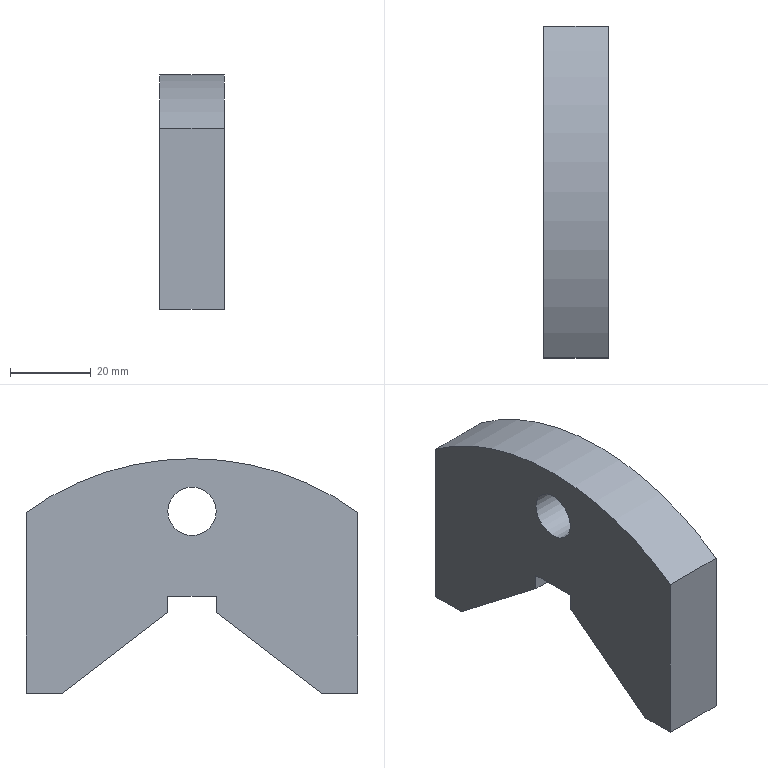Component | NX | V_BLOCK | 1 solid | 13 faces | box 16 x 82 x 58 mm | volume 55776 mm3 | plane 11 | cylinder 2 | commonest cylinder face diameters 140 x1 12 x1
STEP:
#1=CARTESIAN_POINT('',(0.,0.,0.));
#2=DIRECTION('',(0.,0.,1.));
#3=DIRECTION('',(1.,0.,0.));
#4=AXIS2_PLACEMENT_3D('',#1,#2,#3);
#5=CARTESIAN_POINT('',(47.,-41.,189.249));
#6=VERTEX_POINT('',#5);
#7=CARTESIAN_POINT('',(47.,-41.,144.513));
#8=VERTEX_POINT('',#7);
#9=CARTESIAN_POINT('',(47.,-41.,189.249));
#10=DIRECTION('',(0.,-0.,-1.));
#11=VECTOR('',#10,1.);
#12=LINE('',#9,#11);
#13=CARTESIAN_POINT('',(63.,-41.,189.249));
#14=DIRECTION('',(0.,1.,-0.));
#15=DIRECTION('',(0.,0.,1.));
#16=AXIS2_PLACEMENT_3D('',#13,#14,#15);
#17=PLANE('',#16);
#18=CARTESIAN_POINT('',(0.,-16.));
#19=DIRECTION('',(-1.,0.));
#20=VECTOR('',#19,1.);
#21=LINE('',#18,#20);
#22=(GEOMETRIC_REPRESENTATION_CONTEXT(2)PARAMETRIC_REPRESENTATION_CONTEXT()REPRESENTATION_CONTEXT('',''));
#23=DEFINITIONAL_REPRESENTATION('',(#21),#22);
#24=PCURVE('',#17,#23);
#25=CARTESIAN_POINT('',(47.,0.,132.513));
#26=DIRECTION('',(1.,0.,0.));
#27=DIRECTION('',(0.,0.,-1.));
#28=AXIS2_PLACEMENT_3D('',#25,#26,#27);
#29=PLANE('',#28);
#30=CARTESIAN_POINT('',(-56.736,-41.));
#31=DIRECTION('',(1.,-0.));
#32=VECTOR('',#31,1.);
#33=LINE('',#30,#32);
#34=(GEOMETRIC_REPRESENTATION_CONTEXT(2)PARAMETRIC_REPRESENTATION_CONTEXT()REPRESENTATION_CONTEXT('',''));
#35=DEFINITIONAL_REPRESENTATION('',(#33),#34);
#36=PCURVE('',#29,#35);
#37=SURFACE_CURVE('',#12,(#24,#36),.PCURVE_S1.);
#38=EDGE_CURVE('',#6,#8,#37,.T.);
#39=ORIENTED_EDGE('',*,*,#38,.T.);
#40=CARTESIAN_POINT('',(63.,-41.,144.513));
#41=VERTEX_POINT('',#40);
#42=CARTESIAN_POINT('',(63.,-41.,144.513));
#43=DIRECTION('',(-1.,0.,0.));
#44=VECTOR('',#43,1.);
#45=LINE('',#42,#44);
#46=CARTESIAN_POINT('',(-44.736,0.));
#47=DIRECTION('',(0.,-1.));
#48=VECTOR('',#47,1.);
#49=LINE('',#46,#48);
#50=(GEOMETRIC_REPRESENTATION_CONTEXT(2)PARAMETRIC_REPRESENTATION_CONTEXT()REPRESENTATION_CONTEXT('',''));
#51=DEFINITIONAL_REPRESENTATION('',(#49),#50);
#52=PCURVE('',#17,#51);
#53=CARTESIAN_POINT('',(63.,-41.,144.513));
#54=DIRECTION('',(0.,0.,1.));
#55=DIRECTION('',(0.,-1.,0.));
#56=AXIS2_PLACEMENT_3D('',#53,#54,#55);
#57=PLANE('',#56);
#58=CARTESIAN_POINT('',(0.,0.));
#59=DIRECTION('',(0.,-1.));
#60=VECTOR('',#59,1.);
#61=LINE('',#58,#60);
#62=(GEOMETRIC_REPRESENTATION_CONTEXT(2)PARAMETRIC_REPRESENTATION_CONTEXT()REPRESENTATION_CONTEXT('',''));
#63=DEFINITIONAL_REPRESENTATION('',(#61),#62);
#64=PCURVE('',#57,#63);
#65=SURFACE_CURVE('',#45,(#52,#64),.PCURVE_S1.);
#66=EDGE_CURVE('',#41,#8,#65,.T.);
#67=ORIENTED_EDGE('',*,*,#66,.F.);
#68=CARTESIAN_POINT('',(63.,-41.,189.249));
#69=VERTEX_POINT('',#68);
#70=CARTESIAN_POINT('',(63.,-41.,189.249));
#71=DIRECTION('',(0.,-0.,-1.));
#72=VECTOR('',#71,1.);
#73=LINE('',#70,#72);
#74=CARTESIAN_POINT('',(0.,0.));
#75=DIRECTION('',(-1.,0.));
#76=VECTOR('',#75,1.);
#77=LINE('',#74,#76);
#78=(GEOMETRIC_REPRESENTATION_CONTEXT(2)PARAMETRIC_REPRESENTATION_CONTEXT()REPRESENTATION_CONTEXT('',''));
#79=DEFINITIONAL_REPRESENTATION('',(#77),#78);
#80=PCURVE('',#17,#79);
#81=CARTESIAN_POINT('',(63.,0.,132.513));
#82=DIRECTION('',(1.,0.,0.));
#83=DIRECTION('',(0.,0.,-1.));
#84=AXIS2_PLACEMENT_3D('',#81,#82,#83);
#85=PLANE('',#84);
#86=CARTESIAN_POINT('',(-56.736,-41.));
#87=DIRECTION('',(1.,-0.));
#88=VECTOR('',#87,1.);
#89=LINE('',#86,#88);
#90=(GEOMETRIC_REPRESENTATION_CONTEXT(2)PARAMETRIC_REPRESENTATION_CONTEXT()REPRESENTATION_CONTEXT('',''));
#91=DEFINITIONAL_REPRESENTATION('',(#89),#90);
#92=PCURVE('',#85,#91);
#93=SURFACE_CURVE('',#73,(#80,#92),.PCURVE_S1.);
#94=EDGE_CURVE('',#69,#41,#93,.T.);
#95=ORIENTED_EDGE('',*,*,#94,.F.);
#96=CARTESIAN_POINT('',(63.,-41.,189.249));
#97=DIRECTION('',(-1.,0.,0.));
#98=VECTOR('',#97,1.);
#99=LINE('',#96,#98);
#100=CARTESIAN_POINT('',(0.,0.));
#101=DIRECTION('',(0.,-1.));
#102=VECTOR('',#101,1.);
#103=LINE('',#100,#102);
#104=(GEOMETRIC_REPRESENTATION_CONTEXT(2)PARAMETRIC_REPRESENTATION_CONTEXT()REPRESENTATION_CONTEXT('',''));
#105=DEFINITIONAL_REPRESENTATION('',(#103),#104);
#106=PCURVE('',#17,#105);
#107=CARTESIAN_POINT('',(63.,0.,132.513));
#108=DIRECTION('',(-1.,0.,0.));
#109=DIRECTION('',(0.,0.,1.));
#110=AXIS2_PLACEMENT_3D('',#107,#108,#109);
#111=CYLINDRICAL_SURFACE('',#110,70.);
#112=CARTESIAN_POINT('',(-0.6258,0.));
#113=DIRECTION('',(0.,1.));
#114=VECTOR('',#113,1.);
#115=LINE('',#112,#114);
#116=(GEOMETRIC_REPRESENTATION_CONTEXT(2)PARAMETRIC_REPRESENTATION_CONTEXT()REPRESENTATION_CONTEXT('',''));
#117=DEFINITIONAL_REPRESENTATION('',(#115),#116);
#118=PCURVE('',#111,#117);
#119=SURFACE_CURVE('',#99,(#106,#118),.PCURVE_S1.);
#120=EDGE_CURVE('',#69,#6,#119,.T.);
#121=ORIENTED_EDGE('',*,*,#120,.T.);
#122=EDGE_LOOP('',(#39,#67,#95,#121));
#123=FACE_BOUND('',#122,.T.);
#124=ADVANCED_FACE('',(#123),#17,.F.);
#125=CARTESIAN_POINT('',(47.,-32.065,144.513));
#126=VERTEX_POINT('',#125);
#127=CARTESIAN_POINT('',(47.,-41.,144.513));
#128=DIRECTION('',(0.,1.,-0.));
#129=VECTOR('',#128,1.);
#130=LINE('',#127,#129);
#131=CARTESIAN_POINT('',(0.,-16.));
#132=DIRECTION('',(-1.,0.));
#133=VECTOR('',#132,1.);
#134=LINE('',#131,#133);
#135=(GEOMETRIC_REPRESENTATION_CONTEXT(2)PARAMETRIC_REPRESENTATION_CONTEXT()REPRESENTATION_CONTEXT('',''));
#136=DEFINITIONAL_REPRESENTATION('',(#134),#135);
#137=PCURVE('',#57,#136);
#138=CARTESIAN_POINT('',(-12.,-41.));
#139=DIRECTION('',(0.,1.));
#140=VECTOR('',#139,1.);
#141=LINE('',#138,#140);
#142=(GEOMETRIC_REPRESENTATION_CONTEXT(2)PARAMETRIC_REPRESENTATION_CONTEXT()REPRESENTATION_CONTEXT('',''));
#143=DEFINITIONAL_REPRESENTATION('',(#141),#142);
#144=PCURVE('',#29,#143);
#145=SURFACE_CURVE('',#130,(#137,#144),.PCURVE_S1.);
#146=EDGE_CURVE('',#8,#126,#145,.T.);
#147=ORIENTED_EDGE('',*,*,#146,.T.);
#148=CARTESIAN_POINT('',(63.,-32.065,144.513));
#149=VERTEX_POINT('',#148);
#150=CARTESIAN_POINT('',(63.,-32.065,144.513));
#151=DIRECTION('',(-1.,0.,0.));
#152=VECTOR('',#151,1.);
#153=LINE('',#150,#152);
#154=CARTESIAN_POINT('',(-8.935,0.));
#155=DIRECTION('',(0.,-1.));
#156=VECTOR('',#155,1.);
#157=LINE('',#154,#156);
#158=(GEOMETRIC_REPRESENTATION_CONTEXT(2)PARAMETRIC_REPRESENTATION_CONTEXT()REPRESENTATION_CONTEXT('',''));
#159=DEFINITIONAL_REPRESENTATION('',(#157),#158);
#160=PCURVE('',#57,#159);
#161=CARTESIAN_POINT('',(63.,-32.065,144.513));
#162=DIRECTION('',(0.,-0.6088,0.7934));
#163=DIRECTION('',(0.,-0.7934,-0.6088));
#164=AXIS2_PLACEMENT_3D('',#161,#162,#163);
#165=PLANE('',#164);
#166=CARTESIAN_POINT('',(0.,0.));
#167=DIRECTION('',(0.,-1.));
#168=VECTOR('',#167,1.);
#169=LINE('',#166,#168);
#170=(GEOMETRIC_REPRESENTATION_CONTEXT(2)PARAMETRIC_REPRESENTATION_CONTEXT()REPRESENTATION_CONTEXT('',''));
#171=DEFINITIONAL_REPRESENTATION('',(#169),#170);
#172=PCURVE('',#165,#171);
#173=SURFACE_CURVE('',#153,(#160,#172),.PCURVE_S1.);
#174=EDGE_CURVE('',#149,#126,#173,.T.);
#175=ORIENTED_EDGE('',*,*,#174,.F.);
#176=CARTESIAN_POINT('',(63.,-41.,144.513));
#177=DIRECTION('',(0.,1.,-0.));
#178=VECTOR('',#177,1.);
#179=LINE('',#176,#178);
#180=CARTESIAN_POINT('',(0.,0.));
#181=DIRECTION('',(-1.,0.));
#182=VECTOR('',#181,1.);
#183=LINE('',#180,#182);
#184=(GEOMETRIC_REPRESENTATION_CONTEXT(2)PARAMETRIC_REPRESENTATION_CONTEXT()REPRESENTATION_CONTEXT('',''));
#185=DEFINITIONAL_REPRESENTATION('',(#183),#184);
#186=PCURVE('',#57,#185);
#187=CARTESIAN_POINT('',(-12.,-41.));
#188=DIRECTION('',(0.,1.));
#189=VECTOR('',#188,1.);
#190=LINE('',#187,#189);
#191=(GEOMETRIC_REPRESENTATION_CONTEXT(2)PARAMETRIC_REPRESENTATION_CONTEXT()REPRESENTATION_CONTEXT('',''));
#192=DEFINITIONAL_REPRESENTATION('',(#190),#191);
#193=PCURVE('',#85,#192);
#194=SURFACE_CURVE('',#179,(#186,#193),.PCURVE_S1.);
#195=EDGE_CURVE('',#41,#149,#194,.T.);
#196=ORIENTED_EDGE('',*,*,#195,.F.);
#197=ORIENTED_EDGE('',*,*,#66,.T.);
#198=EDGE_LOOP('',(#147,#175,#196,#197));
#199=FACE_BOUND('',#198,.T.);
#200=ADVANCED_FACE('',(#199),#57,.F.);
#201=CARTESIAN_POINT('',(47.,-6.,164.513));
#202=VERTEX_POINT('',#201);
#203=CARTESIAN_POINT('',(47.,-32.065,144.513));
#204=DIRECTION('',(0.,0.7934,0.6088));
#205=VECTOR('',#204,1.);
#206=LINE('',#203,#205);
#207=CARTESIAN_POINT('',(0.,-16.));
#208=DIRECTION('',(-1.,0.));
#209=VECTOR('',#208,1.);
#210=LINE('',#207,#209);
#211=(GEOMETRIC_REPRESENTATION_CONTEXT(2)PARAMETRIC_REPRESENTATION_CONTEXT()REPRESENTATION_CONTEXT('',''));
#212=DEFINITIONAL_REPRESENTATION('',(#210),#211);
#213=PCURVE('',#165,#212);
#214=CARTESIAN_POINT('',(-12.,-32.065));
#215=DIRECTION('',(-0.6088,0.7934));
#216=VECTOR('',#215,1.);
#217=LINE('',#214,#216);
#218=(GEOMETRIC_REPRESENTATION_CONTEXT(2)PARAMETRIC_REPRESENTATION_CONTEXT()REPRESENTATION_CONTEXT('',''));
#219=DEFINITIONAL_REPRESENTATION('',(#217),#218);
#220=PCURVE('',#29,#219);
#221=SURFACE_CURVE('',#206,(#213,#220),.PCURVE_S1.);
#222=EDGE_CURVE('',#126,#202,#221,.T.);
#223=ORIENTED_EDGE('',*,*,#222,.T.);
#224=CARTESIAN_POINT('',(63.,-6.,164.513));
#225=VERTEX_POINT('',#224);
#226=CARTESIAN_POINT('',(63.,-6.,164.513));
#227=DIRECTION('',(-1.,0.,0.));
#228=VECTOR('',#227,1.);
#229=LINE('',#226,#228);
#230=CARTESIAN_POINT('',(-32.854,0.));
#231=DIRECTION('',(0.,-1.));
#232=VECTOR('',#231,1.);
#233=LINE('',#230,#232);
#234=(GEOMETRIC_REPRESENTATION_CONTEXT(2)PARAMETRIC_REPRESENTATION_CONTEXT()REPRESENTATION_CONTEXT('',''));
#235=DEFINITIONAL_REPRESENTATION('',(#233),#234);
#236=PCURVE('',#165,#235);
#237=CARTESIAN_POINT('',(63.,-6.,164.513));
#238=DIRECTION('',(0.,-1.,0.));
#239=DIRECTION('',(0.,0.,-1.));
#240=AXIS2_PLACEMENT_3D('',#237,#238,#239);
#241=PLANE('',#240);
#242=CARTESIAN_POINT('',(0.,0.));
#243=DIRECTION('',(0.,-1.));
#244=VECTOR('',#243,1.);
#245=LINE('',#242,#244);
#246=(GEOMETRIC_REPRESENTATION_CONTEXT(2)PARAMETRIC_REPRESENTATION_CONTEXT()REPRESENTATION_CONTEXT('',''));
#247=DEFINITIONAL_REPRESENTATION('',(#245),#246);
#248=PCURVE('',#241,#247);
#249=SURFACE_CURVE('',#229,(#236,#248),.PCURVE_S1.);
#250=EDGE_CURVE('',#225,#202,#249,.T.);
#251=ORIENTED_EDGE('',*,*,#250,.F.);
#252=CARTESIAN_POINT('',(63.,-32.065,144.513));
#253=DIRECTION('',(0.,0.7934,0.6088));
#254=VECTOR('',#253,1.);
#255=LINE('',#252,#254);
#256=CARTESIAN_POINT('',(0.,0.));
#257=DIRECTION('',(-1.,0.));
#258=VECTOR('',#257,1.);
#259=LINE('',#256,#258);
#260=(GEOMETRIC_REPRESENTATION_CONTEXT(2)PARAMETRIC_REPRESENTATION_CONTEXT()REPRESENTATION_CONTEXT('',''));
#261=DEFINITIONAL_REPRESENTATION('',(#259),#260);
#262=PCURVE('',#165,#261);
#263=CARTESIAN_POINT('',(-12.,-32.065));
#264=DIRECTION('',(-0.6088,0.7934));
#265=VECTOR('',#264,1.);
#266=LINE('',#263,#265);
#267=(GEOMETRIC_REPRESENTATION_CONTEXT(2)PARAMETRIC_REPRESENTATION_CONTEXT()REPRESENTATION_CONTEXT('',''));
#268=DEFINITIONAL_REPRESENTATION('',(#266),#267);
#269=PCURVE('',#85,#268);
#270=SURFACE_CURVE('',#255,(#262,#269),.PCURVE_S1.);
#271=EDGE_CURVE('',#149,#225,#270,.T.);
#272=ORIENTED_EDGE('',*,*,#271,.F.);
#273=ORIENTED_EDGE('',*,*,#174,.T.);
#274=EDGE_LOOP('',(#223,#251,#272,#273));
#275=FACE_BOUND('',#274,.T.);
#276=ADVANCED_FACE('',(#275),#165,.F.);
#277=CARTESIAN_POINT('',(47.,-6.,168.513));
#278=VERTEX_POINT('',#277);
#279=CARTESIAN_POINT('',(47.,-6.,164.513));
#280=DIRECTION('',(0.,0.,1.));
#281=VECTOR('',#280,1.);
#282=LINE('',#279,#281);
#283=CARTESIAN_POINT('',(0.,-16.));
#284=DIRECTION('',(-1.,0.));
#285=VECTOR('',#284,1.);
#286=LINE('',#283,#285);
#287=(GEOMETRIC_REPRESENTATION_CONTEXT(2)PARAMETRIC_REPRESENTATION_CONTEXT()REPRESENTATION_CONTEXT('',''));
#288=DEFINITIONAL_REPRESENTATION('',(#286),#287);
#289=PCURVE('',#241,#288);
#290=CARTESIAN_POINT('',(-32.,-6.));
#291=DIRECTION('',(-1.,0.));
#292=VECTOR('',#291,1.);
#293=LINE('',#290,#292);
#294=(GEOMETRIC_REPRESENTATION_CONTEXT(2)PARAMETRIC_REPRESENTATION_CONTEXT()REPRESENTATION_CONTEXT('',''));
#295=DEFINITIONAL_REPRESENTATION('',(#293),#294);
#296=PCURVE('',#29,#295);
#297=SURFACE_CURVE('',#282,(#289,#296),.PCURVE_S1.);
#298=EDGE_CURVE('',#202,#278,#297,.T.);
#299=ORIENTED_EDGE('',*,*,#298,.T.);
#300=CARTESIAN_POINT('',(63.,-6.,168.513));
#301=VERTEX_POINT('',#300);
#302=CARTESIAN_POINT('',(63.,-6.,168.513));
#303=DIRECTION('',(-1.,0.,0.));
#304=VECTOR('',#303,1.);
#305=LINE('',#302,#304);
#306=CARTESIAN_POINT('',(-4.,0.));
#307=DIRECTION('',(0.,-1.));
#308=VECTOR('',#307,1.);
#309=LINE('',#306,#308);
#310=(GEOMETRIC_REPRESENTATION_CONTEXT(2)PARAMETRIC_REPRESENTATION_CONTEXT()REPRESENTATION_CONTEXT('',''));
#311=DEFINITIONAL_REPRESENTATION('',(#309),#310);
#312=PCURVE('',#241,#311);
#313=CARTESIAN_POINT('',(63.,0.,168.513));
#314=DIRECTION('',(0.,0.,1.));
#315=DIRECTION('',(1.,0.,0.));
#316=AXIS2_PLACEMENT_3D('',#313,#314,#315);
#317=PLANE('',#316);
#318=CARTESIAN_POINT('',(0.,-6.));
#319=DIRECTION('',(-1.,0.));
#320=VECTOR('',#319,1.);
#321=LINE('',#318,#320);
#322=(GEOMETRIC_REPRESENTATION_CONTEXT(2)PARAMETRIC_REPRESENTATION_CONTEXT()REPRESENTATION_CONTEXT('',''));
#323=DEFINITIONAL_REPRESENTATION('',(#321),#322);
#324=PCURVE('',#317,#323);
#325=SURFACE_CURVE('',#305,(#312,#324),.PCURVE_S1.);
#326=EDGE_CURVE('',#301,#278,#325,.T.);
#327=ORIENTED_EDGE('',*,*,#326,.F.);
#328=CARTESIAN_POINT('',(63.,-6.,164.513));
#329=DIRECTION('',(0.,0.,1.));
#330=VECTOR('',#329,1.);
#331=LINE('',#328,#330);
#332=CARTESIAN_POINT('',(0.,0.));
#333=DIRECTION('',(-1.,0.));
#334=VECTOR('',#333,1.);
#335=LINE('',#332,#334);
#336=(GEOMETRIC_REPRESENTATION_CONTEXT(2)PARAMETRIC_REPRESENTATION_CONTEXT()REPRESENTATION_CONTEXT('',''));
#337=DEFINITIONAL_REPRESENTATION('',(#335),#336);
#338=PCURVE('',#241,#337);
#339=CARTESIAN_POINT('',(-32.,-6.));
#340=DIRECTION('',(-1.,0.));
#341=VECTOR('',#340,1.);
#342=LINE('',#339,#341);
#343=(GEOMETRIC_REPRESENTATION_CONTEXT(2)PARAMETRIC_REPRESENTATION_CONTEXT()REPRESENTATION_CONTEXT('',''));
#344=DEFINITIONAL_REPRESENTATION('',(#342),#343);
#345=PCURVE('',#85,#344);
#346=SURFACE_CURVE('',#331,(#338,#345),.PCURVE_S1.);
#347=EDGE_CURVE('',#225,#301,#346,.T.);
#348=ORIENTED_EDGE('',*,*,#347,.F.);
#349=ORIENTED_EDGE('',*,*,#250,.T.);
#350=EDGE_LOOP('',(#299,#327,#348,#349));
#351=FACE_BOUND('',#350,.T.);
#352=ADVANCED_FACE('',(#351),#241,.F.);
#353=CARTESIAN_POINT('',(47.,6.,168.513));
#354=VERTEX_POINT('',#353);
#355=CARTESIAN_POINT('',(47.,0.,168.513));
#356=DIRECTION('',(0.,1.,0.));
#357=VECTOR('',#356,1.);
#358=LINE('',#355,#357);
#359=CARTESIAN_POINT('',(-16.,0.));
#360=DIRECTION('',(0.,1.));
#361=VECTOR('',#360,1.);
#362=LINE('',#359,#361);
#363=(GEOMETRIC_REPRESENTATION_CONTEXT(2)PARAMETRIC_REPRESENTATION_CONTEXT()REPRESENTATION_CONTEXT('',''));
#364=DEFINITIONAL_REPRESENTATION('',(#362),#363);
#365=PCURVE('',#317,#364);
#366=CARTESIAN_POINT('',(-36.,0.));
#367=DIRECTION('',(0.,1.));
#368=VECTOR('',#367,1.);
#369=LINE('',#366,#368);
#370=(GEOMETRIC_REPRESENTATION_CONTEXT(2)PARAMETRIC_REPRESENTATION_CONTEXT()REPRESENTATION_CONTEXT('',''));
#371=DEFINITIONAL_REPRESENTATION('',(#369),#370);
#372=PCURVE('',#29,#371);
#373=SURFACE_CURVE('',#358,(#365,#372),.PCURVE_S1.);
#374=EDGE_CURVE('',#278,#354,#373,.T.);
#375=ORIENTED_EDGE('',*,*,#374,.T.);
#376=CARTESIAN_POINT('',(63.,6.,168.513));
#377=VERTEX_POINT('',#376);
#378=CARTESIAN_POINT('',(63.,6.,168.513));
#379=DIRECTION('',(-1.,0.,0.));
#380=VECTOR('',#379,1.);
#381=LINE('',#378,#380);
#382=CARTESIAN_POINT('',(0.,6.));
#383=DIRECTION('',(-1.,0.));
#384=VECTOR('',#383,1.);
#385=LINE('',#382,#384);
#386=(GEOMETRIC_REPRESENTATION_CONTEXT(2)PARAMETRIC_REPRESENTATION_CONTEXT()REPRESENTATION_CONTEXT('',''));
#387=DEFINITIONAL_REPRESENTATION('',(#385),#386);
#388=PCURVE('',#317,#387);
#389=CARTESIAN_POINT('',(63.,6.,168.513));
#390=DIRECTION('',(0.,1.,0.));
#391=DIRECTION('',(0.,0.,1.));
#392=AXIS2_PLACEMENT_3D('',#389,#390,#391);
#393=PLANE('',#392);
#394=CARTESIAN_POINT('',(0.,0.));
#395=DIRECTION('',(0.,-1.));
#396=VECTOR('',#395,1.);
#397=LINE('',#394,#396);
#398=(GEOMETRIC_REPRESENTATION_CONTEXT(2)PARAMETRIC_REPRESENTATION_CONTEXT()REPRESENTATION_CONTEXT('',''));
#399=DEFINITIONAL_REPRESENTATION('',(#397),#398);
#400=PCURVE('',#393,#399);
#401=SURFACE_CURVE('',#381,(#388,#400),.PCURVE_S1.);
#402=EDGE_CURVE('',#377,#354,#401,.T.);
#403=ORIENTED_EDGE('',*,*,#402,.F.);
#404=CARTESIAN_POINT('',(63.,-6.,168.513));
#405=DIRECTION('',(0.,1.,0.));
#406=VECTOR('',#405,1.);
#407=LINE('',#404,#406);
#408=CARTESIAN_POINT('',(0.,-6.));
#409=DIRECTION('',(0.,1.));
#410=VECTOR('',#409,1.);
#411=LINE('',#408,#410);
#412=(GEOMETRIC_REPRESENTATION_CONTEXT(2)PARAMETRIC_REPRESENTATION_CONTEXT()REPRESENTATION_CONTEXT('',''));
#413=DEFINITIONAL_REPRESENTATION('',(#411),#412);
#414=PCURVE('',#317,#413);
#415=CARTESIAN_POINT('',(-36.,-6.));
#416=DIRECTION('',(0.,1.));
#417=VECTOR('',#416,1.);
#418=LINE('',#415,#417);
#419=(GEOMETRIC_REPRESENTATION_CONTEXT(2)PARAMETRIC_REPRESENTATION_CONTEXT()REPRESENTATION_CONTEXT('',''));
#420=DEFINITIONAL_REPRESENTATION('',(#418),#419);
#421=PCURVE('',#85,#420);
#422=SURFACE_CURVE('',#407,(#414,#421),.PCURVE_S1.);
#423=EDGE_CURVE('',#301,#377,#422,.T.);
#424=ORIENTED_EDGE('',*,*,#423,.F.);
#425=ORIENTED_EDGE('',*,*,#326,.T.);
#426=EDGE_LOOP('',(#375,#403,#424,#425));
#427=FACE_BOUND('',#426,.T.);
#428=ADVANCED_FACE('',(#427),#317,.F.);
#429=CARTESIAN_POINT('',(47.,6.,164.513));
#430=VERTEX_POINT('',#429);
#431=CARTESIAN_POINT('',(47.,6.,168.513));
#432=DIRECTION('',(0.,0.,-1.));
#433=VECTOR('',#432,1.);
#434=LINE('',#431,#433);
#435=CARTESIAN_POINT('',(0.,-16.));
#436=DIRECTION('',(-1.,0.));
#437=VECTOR('',#436,1.);
#438=LINE('',#435,#437);
#439=(GEOMETRIC_REPRESENTATION_CONTEXT(2)PARAMETRIC_REPRESENTATION_CONTEXT()REPRESENTATION_CONTEXT('',''));
#440=DEFINITIONAL_REPRESENTATION('',(#438),#439);
#441=PCURVE('',#393,#440);
#442=CARTESIAN_POINT('',(-36.,6.));
#443=DIRECTION('',(1.,0.));
#444=VECTOR('',#443,1.);
#445=LINE('',#442,#444);
#446=(GEOMETRIC_REPRESENTATION_CONTEXT(2)PARAMETRIC_REPRESENTATION_CONTEXT()REPRESENTATION_CONTEXT('',''));
#447=DEFINITIONAL_REPRESENTATION('',(#445),#446);
#448=PCURVE('',#29,#447);
#449=SURFACE_CURVE('',#434,(#441,#448),.PCURVE_S1.);
#450=EDGE_CURVE('',#354,#430,#449,.T.);
#451=ORIENTED_EDGE('',*,*,#450,.T.);
#452=CARTESIAN_POINT('',(63.,6.,164.513));
#453=VERTEX_POINT('',#452);
#454=CARTESIAN_POINT('',(63.,6.,164.513));
#455=DIRECTION('',(-1.,0.,0.));
#456=VECTOR('',#455,1.);
#457=LINE('',#454,#456);
#458=CARTESIAN_POINT('',(-4.,0.));
#459=DIRECTION('',(0.,-1.));
#460=VECTOR('',#459,1.);
#461=LINE('',#458,#460);
#462=(GEOMETRIC_REPRESENTATION_CONTEXT(2)PARAMETRIC_REPRESENTATION_CONTEXT()REPRESENTATION_CONTEXT('',''));
#463=DEFINITIONAL_REPRESENTATION('',(#461),#462);
#464=PCURVE('',#393,#463);
#465=CARTESIAN_POINT('',(63.,6.,164.513));
#466=DIRECTION('',(0.,0.6088,0.7934));
#467=DIRECTION('',(0.,-0.7934,0.6088));
#468=AXIS2_PLACEMENT_3D('',#465,#466,#467);
#469=PLANE('',#468);
#470=CARTESIAN_POINT('',(0.,0.));
#471=DIRECTION('',(0.,-1.));
#472=VECTOR('',#471,1.);
#473=LINE('',#470,#472);
#474=(GEOMETRIC_REPRESENTATION_CONTEXT(2)PARAMETRIC_REPRESENTATION_CONTEXT()REPRESENTATION_CONTEXT('',''));
#475=DEFINITIONAL_REPRESENTATION('',(#473),#474);
#476=PCURVE('',#469,#475);
#477=SURFACE_CURVE('',#457,(#464,#476),.PCURVE_S1.);
#478=EDGE_CURVE('',#453,#430,#477,.T.);
#479=ORIENTED_EDGE('',*,*,#478,.F.);
#480=CARTESIAN_POINT('',(63.,6.,168.513));
#481=DIRECTION('',(0.,0.,-1.));
#482=VECTOR('',#481,1.);
#483=LINE('',#480,#482);
#484=CARTESIAN_POINT('',(0.,0.));
#485=DIRECTION('',(-1.,0.));
#486=VECTOR('',#485,1.);
#487=LINE('',#484,#486);
#488=(GEOMETRIC_REPRESENTATION_CONTEXT(2)PARAMETRIC_REPRESENTATION_CONTEXT()REPRESENTATION_CONTEXT('',''));
#489=DEFINITIONAL_REPRESENTATION('',(#487),#488);
#490=PCURVE('',#393,#489);
#491=CARTESIAN_POINT('',(-36.,6.));
#492=DIRECTION('',(1.,0.));
#493=VECTOR('',#492,1.);
#494=LINE('',#491,#493);
#495=(GEOMETRIC_REPRESENTATION_CONTEXT(2)PARAMETRIC_REPRESENTATION_CONTEXT()REPRESENTATION_CONTEXT('',''));
#496=DEFINITIONAL_REPRESENTATION('',(#494),#495);
#497=PCURVE('',#85,#496);
#498=SURFACE_CURVE('',#483,(#490,#497),.PCURVE_S1.);
#499=EDGE_CURVE('',#377,#453,#498,.T.);
#500=ORIENTED_EDGE('',*,*,#499,.F.);
#501=ORIENTED_EDGE('',*,*,#402,.T.);
#502=EDGE_LOOP('',(#451,#479,#500,#501));
#503=FACE_BOUND('',#502,.T.);
#504=ADVANCED_FACE('',(#503),#393,.F.);
#505=CARTESIAN_POINT('',(47.,32.065,144.513));
#506=VERTEX_POINT('',#505);
#507=CARTESIAN_POINT('',(47.,6.,164.513));
#508=DIRECTION('',(0.,0.7934,-0.6088));
#509=VECTOR('',#508,1.);
#510=LINE('',#507,#509);
#511=CARTESIAN_POINT('',(0.,-16.));
#512=DIRECTION('',(-1.,0.));
#513=VECTOR('',#512,1.);
#514=LINE('',#511,#513);
#515=(GEOMETRIC_REPRESENTATION_CONTEXT(2)PARAMETRIC_REPRESENTATION_CONTEXT()REPRESENTATION_CONTEXT('',''));
#516=DEFINITIONAL_REPRESENTATION('',(#514),#515);
#517=PCURVE('',#469,#516);
#518=CARTESIAN_POINT('',(-32.,6.));
#519=DIRECTION('',(0.6088,0.7934));
#520=VECTOR('',#519,1.);
#521=LINE('',#518,#520);
#522=(GEOMETRIC_REPRESENTATION_CONTEXT(2)PARAMETRIC_REPRESENTATION_CONTEXT()REPRESENTATION_CONTEXT('',''));
#523=DEFINITIONAL_REPRESENTATION('',(#521),#522);
#524=PCURVE('',#29,#523);
#525=SURFACE_CURVE('',#510,(#517,#524),.PCURVE_S1.);
#526=EDGE_CURVE('',#430,#506,#525,.T.);
#527=ORIENTED_EDGE('',*,*,#526,.T.);
#528=CARTESIAN_POINT('',(63.,32.065,144.513));
#529=VERTEX_POINT('',#528);
#530=CARTESIAN_POINT('',(63.,32.065,144.513));
#531=DIRECTION('',(-1.,0.,0.));
#532=VECTOR('',#531,1.);
#533=LINE('',#530,#532);
#534=CARTESIAN_POINT('',(-32.854,0.));
#535=DIRECTION('',(0.,-1.));
#536=VECTOR('',#535,1.);
#537=LINE('',#534,#536);
#538=(GEOMETRIC_REPRESENTATION_CONTEXT(2)PARAMETRIC_REPRESENTATION_CONTEXT()REPRESENTATION_CONTEXT('',''));
#539=DEFINITIONAL_REPRESENTATION('',(#537),#538);
#540=PCURVE('',#469,#539);
#541=CARTESIAN_POINT('',(63.,32.065,144.513));
#542=DIRECTION('',(0.,-0.,1.));
#543=DIRECTION('',(0.,-1.,-0.));
#544=AXIS2_PLACEMENT_3D('',#541,#542,#543);
#545=PLANE('',#544);
#546=CARTESIAN_POINT('',(0.,0.));
#547=DIRECTION('',(0.,-1.));
#548=VECTOR('',#547,1.);
#549=LINE('',#546,#548);
#550=(GEOMETRIC_REPRESENTATION_CONTEXT(2)PARAMETRIC_REPRESENTATION_CONTEXT()REPRESENTATION_CONTEXT('',''));
#551=DEFINITIONAL_REPRESENTATION('',(#549),#550);
#552=PCURVE('',#545,#551);
#553=SURFACE_CURVE('',#533,(#540,#552),.PCURVE_S1.);
#554=EDGE_CURVE('',#529,#506,#553,.T.);
#555=ORIENTED_EDGE('',*,*,#554,.F.);
#556=CARTESIAN_POINT('',(63.,6.,164.513));
#557=DIRECTION('',(0.,0.7934,-0.6088));
#558=VECTOR('',#557,1.);
#559=LINE('',#556,#558);
#560=CARTESIAN_POINT('',(0.,0.));
#561=DIRECTION('',(-1.,0.));
#562=VECTOR('',#561,1.);
#563=LINE('',#560,#562);
#564=(GEOMETRIC_REPRESENTATION_CONTEXT(2)PARAMETRIC_REPRESENTATION_CONTEXT()REPRESENTATION_CONTEXT('',''));
#565=DEFINITIONAL_REPRESENTATION('',(#563),#564);
#566=PCURVE('',#469,#565);
#567=CARTESIAN_POINT('',(-32.,6.));
#568=DIRECTION('',(0.6088,0.7934));
#569=VECTOR('',#568,1.);
#570=LINE('',#567,#569);
#571=(GEOMETRIC_REPRESENTATION_CONTEXT(2)PARAMETRIC_REPRESENTATION_CONTEXT()REPRESENTATION_CONTEXT('',''));
#572=DEFINITIONAL_REPRESENTATION('',(#570),#571);
#573=PCURVE('',#85,#572);
#574=SURFACE_CURVE('',#559,(#566,#573),.PCURVE_S1.);
#575=EDGE_CURVE('',#453,#529,#574,.T.);
#576=ORIENTED_EDGE('',*,*,#575,.F.);
#577=ORIENTED_EDGE('',*,*,#478,.T.);
#578=EDGE_LOOP('',(#527,#555,#576,#577));
#579=FACE_BOUND('',#578,.T.);
#580=ADVANCED_FACE('',(#579),#469,.F.);
#581=CARTESIAN_POINT('',(47.,41.,144.513));
#582=VERTEX_POINT('',#581);
#583=CARTESIAN_POINT('',(47.,32.065,144.513));
#584=DIRECTION('',(0.,1.,0.));
#585=VECTOR('',#584,1.);
#586=LINE('',#583,#585);
#587=CARTESIAN_POINT('',(0.,-16.));
#588=DIRECTION('',(-1.,0.));
#589=VECTOR('',#588,1.);
#590=LINE('',#587,#589);
#591=(GEOMETRIC_REPRESENTATION_CONTEXT(2)PARAMETRIC_REPRESENTATION_CONTEXT()REPRESENTATION_CONTEXT('',''));
#592=DEFINITIONAL_REPRESENTATION('',(#590),#591);
#593=PCURVE('',#545,#592);
#594=CARTESIAN_POINT('',(-12.,32.065));
#595=DIRECTION('',(-0.,1.));
#596=VECTOR('',#595,1.);
#597=LINE('',#594,#596);
#598=(GEOMETRIC_REPRESENTATION_CONTEXT(2)PARAMETRIC_REPRESENTATION_CONTEXT()REPRESENTATION_CONTEXT('',''));
#599=DEFINITIONAL_REPRESENTATION('',(#597),#598);
#600=PCURVE('',#29,#599);
#601=SURFACE_CURVE('',#586,(#593,#600),.PCURVE_S1.);
#602=EDGE_CURVE('',#506,#582,#601,.T.);
#603=ORIENTED_EDGE('',*,*,#602,.T.);
#604=CARTESIAN_POINT('',(63.,41.,144.513));
#605=VERTEX_POINT('',#604);
#606=CARTESIAN_POINT('',(63.,41.,144.513));
#607=DIRECTION('',(-1.,0.,0.));
#608=VECTOR('',#607,1.);
#609=LINE('',#606,#608);
#610=CARTESIAN_POINT('',(-8.935,0.));
#611=DIRECTION('',(0.,-1.));
#612=VECTOR('',#611,1.);
#613=LINE('',#610,#612);
#614=(GEOMETRIC_REPRESENTATION_CONTEXT(2)PARAMETRIC_REPRESENTATION_CONTEXT()REPRESENTATION_CONTEXT('',''));
#615=DEFINITIONAL_REPRESENTATION('',(#613),#614);
#616=PCURVE('',#545,#615);
#617=CARTESIAN_POINT('',(63.,41.,144.513));
#618=DIRECTION('',(0.,-1.,-0.));
#619=DIRECTION('',(0.,0.,-1.));
#620=AXIS2_PLACEMENT_3D('',#617,#618,#619);
#621=PLANE('',#620);
#622=CARTESIAN_POINT('',(0.,0.));
#623=DIRECTION('',(0.,-1.));
#624=VECTOR('',#623,1.);
#625=LINE('',#622,#624);
#626=(GEOMETRIC_REPRESENTATION_CONTEXT(2)PARAMETRIC_REPRESENTATION_CONTEXT()REPRESENTATION_CONTEXT('',''));
#627=DEFINITIONAL_REPRESENTATION('',(#625),#626);
#628=PCURVE('',#621,#627);
#629=SURFACE_CURVE('',#609,(#616,#628),.PCURVE_S1.);
#630=EDGE_CURVE('',#605,#582,#629,.T.);
#631=ORIENTED_EDGE('',*,*,#630,.F.);
#632=CARTESIAN_POINT('',(63.,32.065,144.513));
#633=DIRECTION('',(0.,1.,0.));
#634=VECTOR('',#633,1.);
#635=LINE('',#632,#634);
#636=CARTESIAN_POINT('',(0.,0.));
#637=DIRECTION('',(-1.,0.));
#638=VECTOR('',#637,1.);
#639=LINE('',#636,#638);
#640=(GEOMETRIC_REPRESENTATION_CONTEXT(2)PARAMETRIC_REPRESENTATION_CONTEXT()REPRESENTATION_CONTEXT('',''));
#641=DEFINITIONAL_REPRESENTATION('',(#639),#640);
#642=PCURVE('',#545,#641);
#643=CARTESIAN_POINT('',(-12.,32.065));
#644=DIRECTION('',(-0.,1.));
#645=VECTOR('',#644,1.);
#646=LINE('',#643,#645);
#647=(GEOMETRIC_REPRESENTATION_CONTEXT(2)PARAMETRIC_REPRESENTATION_CONTEXT()REPRESENTATION_CONTEXT('',''));
#648=DEFINITIONAL_REPRESENTATION('',(#646),#647);
#649=PCURVE('',#85,#648);
#650=SURFACE_CURVE('',#635,(#642,#649),.PCURVE_S1.);
#651=EDGE_CURVE('',#529,#605,#650,.T.);
#652=ORIENTED_EDGE('',*,*,#651,.F.);
#653=ORIENTED_EDGE('',*,*,#554,.T.);
#654=EDGE_LOOP('',(#603,#631,#652,#653));
#655=FACE_BOUND('',#654,.T.);
#656=ADVANCED_FACE('',(#655),#545,.F.);
#657=CARTESIAN_POINT('',(47.,41.,189.249));
#658=VERTEX_POINT('',#657);
#659=CARTESIAN_POINT('',(47.,41.,144.513));
#660=DIRECTION('',(0.,-0.,1.));
#661=VECTOR('',#660,1.);
#662=LINE('',#659,#661);
#663=CARTESIAN_POINT('',(0.,-16.));
#664=DIRECTION('',(-1.,0.));
#665=VECTOR('',#664,1.);
#666=LINE('',#663,#665);
#667=(GEOMETRIC_REPRESENTATION_CONTEXT(2)PARAMETRIC_REPRESENTATION_CONTEXT()REPRESENTATION_CONTEXT('',''));
#668=DEFINITIONAL_REPRESENTATION('',(#666),#667);
#669=PCURVE('',#621,#668);
#670=CARTESIAN_POINT('',(-12.,41.));
#671=DIRECTION('',(-1.,-0.));
#672=VECTOR('',#671,1.);
#673=LINE('',#670,#672);
#674=(GEOMETRIC_REPRESENTATION_CONTEXT(2)PARAMETRIC_REPRESENTATION_CONTEXT()REPRESENTATION_CONTEXT('',''));
#675=DEFINITIONAL_REPRESENTATION('',(#673),#674);
#676=PCURVE('',#29,#675);
#677=SURFACE_CURVE('',#662,(#669,#676),.PCURVE_S1.);
#678=EDGE_CURVE('',#582,#658,#677,.T.);
#679=ORIENTED_EDGE('',*,*,#678,.T.);
#680=CARTESIAN_POINT('',(63.,41.,189.249));
#681=VERTEX_POINT('',#680);
#682=CARTESIAN_POINT('',(63.,41.,189.249));
#683=DIRECTION('',(-1.,0.,0.));
#684=VECTOR('',#683,1.);
#685=LINE('',#682,#684);
#686=CARTESIAN_POINT('',(-44.736,0.));
#687=DIRECTION('',(0.,-1.));
#688=VECTOR('',#687,1.);
#689=LINE('',#686,#688);
#690=(GEOMETRIC_REPRESENTATION_CONTEXT(2)PARAMETRIC_REPRESENTATION_CONTEXT()REPRESENTATION_CONTEXT('',''));
#691=DEFINITIONAL_REPRESENTATION('',(#689),#690);
#692=PCURVE('',#621,#691);
#693=CARTESIAN_POINT('',(0.6258,0.));
#694=DIRECTION('',(0.,1.));
#695=VECTOR('',#694,1.);
#696=LINE('',#693,#695);
#697=(GEOMETRIC_REPRESENTATION_CONTEXT(2)PARAMETRIC_REPRESENTATION_CONTEXT()REPRESENTATION_CONTEXT('',''));
#698=DEFINITIONAL_REPRESENTATION('',(#696),#697);
#699=PCURVE('',#111,#698);
#700=SURFACE_CURVE('',#685,(#692,#699),.PCURVE_S1.);
#701=EDGE_CURVE('',#681,#658,#700,.T.);
#702=ORIENTED_EDGE('',*,*,#701,.F.);
#703=CARTESIAN_POINT('',(63.,41.,144.513));
#704=DIRECTION('',(0.,-0.,1.));
#705=VECTOR('',#704,1.);
#706=LINE('',#703,#705);
#707=CARTESIAN_POINT('',(0.,0.));
#708=DIRECTION('',(-1.,0.));
#709=VECTOR('',#708,1.);
#710=LINE('',#707,#709);
#711=(GEOMETRIC_REPRESENTATION_CONTEXT(2)PARAMETRIC_REPRESENTATION_CONTEXT()REPRESENTATION_CONTEXT('',''));
#712=DEFINITIONAL_REPRESENTATION('',(#710),#711);
#713=PCURVE('',#621,#712);
#714=CARTESIAN_POINT('',(-12.,41.));
#715=DIRECTION('',(-1.,-0.));
#716=VECTOR('',#715,1.);
#717=LINE('',#714,#716);
#718=(GEOMETRIC_REPRESENTATION_CONTEXT(2)PARAMETRIC_REPRESENTATION_CONTEXT()REPRESENTATION_CONTEXT('',''));
#719=DEFINITIONAL_REPRESENTATION('',(#717),#718);
#720=PCURVE('',#85,#719);
#721=SURFACE_CURVE('',#706,(#713,#720),.PCURVE_S1.);
#722=EDGE_CURVE('',#605,#681,#721,.T.);
#723=ORIENTED_EDGE('',*,*,#722,.F.);
#724=ORIENTED_EDGE('',*,*,#630,.T.);
#725=EDGE_LOOP('',(#679,#702,#723,#724));
#726=FACE_BOUND('',#725,.T.);
#727=ADVANCED_FACE('',(#726),#621,.F.);
#728=CARTESIAN_POINT('',(47.,0.,132.513));
#729=DIRECTION('',(1.,0.,0.));
#730=DIRECTION('',(0.,1.,0.));
#731=AXIS2_PLACEMENT_3D('',#728,#729,#730);
#732=CIRCLE('',#731,70.);
#733=CARTESIAN_POINT('',(1.571,16.));
#734=DIRECTION('',(-1.,0.));
#735=VECTOR('',#734,1.);
#736=LINE('',#733,#735);
#737=(GEOMETRIC_REPRESENTATION_CONTEXT(2)PARAMETRIC_REPRESENTATION_CONTEXT()REPRESENTATION_CONTEXT('',''));
#738=DEFINITIONAL_REPRESENTATION('',(#736),#737);
#739=PCURVE('',#111,#738);
#740=CARTESIAN_POINT('',(0.,0.));
#741=DIRECTION('',(0.,1.));
#742=AXIS2_PLACEMENT_2D('',#740,#741);
#743=CIRCLE('',#742,70.);
#744=(GEOMETRIC_REPRESENTATION_CONTEXT(2)PARAMETRIC_REPRESENTATION_CONTEXT()REPRESENTATION_CONTEXT('',''));
#745=DEFINITIONAL_REPRESENTATION('',(#743),#744);
#746=PCURVE('',#29,#745);
#747=SURFACE_CURVE('',#732,(#739,#746),.PCURVE_S1.);
#748=EDGE_CURVE('',#658,#6,#747,.T.);
#749=ORIENTED_EDGE('',*,*,#748,.T.);
#750=ORIENTED_EDGE('',*,*,#120,.F.);
#751=CARTESIAN_POINT('',(63.,0.,132.513));
#752=DIRECTION('',(1.,0.,0.));
#753=DIRECTION('',(0.,-1.,0.));
#754=AXIS2_PLACEMENT_3D('',#751,#752,#753);
#755=CIRCLE('',#754,70.);
#756=CARTESIAN_POINT('',(4.712,0.));
#757=DIRECTION('',(-1.,0.));
#758=VECTOR('',#757,1.);
#759=LINE('',#756,#758);
#760=(GEOMETRIC_REPRESENTATION_CONTEXT(2)PARAMETRIC_REPRESENTATION_CONTEXT()REPRESENTATION_CONTEXT('',''));
#761=DEFINITIONAL_REPRESENTATION('',(#759),#760);
#762=PCURVE('',#111,#761);
#763=CARTESIAN_POINT('',(0.,0.));
#764=DIRECTION('',(0.,-1.));
#765=AXIS2_PLACEMENT_2D('',#763,#764);
#766=CIRCLE('',#765,70.);
#767=(GEOMETRIC_REPRESENTATION_CONTEXT(2)PARAMETRIC_REPRESENTATION_CONTEXT()REPRESENTATION_CONTEXT('',''));
#768=DEFINITIONAL_REPRESENTATION('',(#766),#767);
#769=PCURVE('',#85,#768);
#770=SURFACE_CURVE('',#755,(#762,#769),.PCURVE_S1.);
#771=EDGE_CURVE('',#681,#69,#770,.T.);
#772=ORIENTED_EDGE('',*,*,#771,.F.);
#773=ORIENTED_EDGE('',*,*,#701,.T.);
#774=EDGE_LOOP('',(#749,#750,#772,#773));
#775=FACE_BOUND('',#774,.T.);
#776=ADVANCED_FACE('',(#775),#111,.T.);
#777=CARTESIAN_POINT('',(63.,6.,189.513));
#778=VERTEX_POINT('',#777);
#779=CARTESIAN_POINT('',(63.,0.,189.513));
#780=DIRECTION('',(1.,0.,0.));
#781=DIRECTION('',(0.,1.,0.));
#782=AXIS2_PLACEMENT_3D('',#779,#780,#781);
#783=CIRCLE('',#782,6.);
#784=CARTESIAN_POINT('',(-57.,0.));
#785=DIRECTION('',(0.,1.));
#786=AXIS2_PLACEMENT_2D('',#784,#785);
#787=CIRCLE('',#786,6.);
#788=(GEOMETRIC_REPRESENTATION_CONTEXT(2)PARAMETRIC_REPRESENTATION_CONTEXT()REPRESENTATION_CONTEXT('',''));
#789=DEFINITIONAL_REPRESENTATION('',(#787),#788);
#790=PCURVE('',#85,#789);
#791=CARTESIAN_POINT('',(63.,0.,189.513));
#792=DIRECTION('',(-1.,0.,0.));
#793=DIRECTION('',(0.,0.,1.));
#794=AXIS2_PLACEMENT_3D('',#791,#792,#793);
#795=CYLINDRICAL_SURFACE('',#794,6.);
#796=CARTESIAN_POINT('',(7.854,0.));
#797=DIRECTION('',(-1.,0.));
#798=VECTOR('',#797,1.);
#799=LINE('',#796,#798);
#800=(GEOMETRIC_REPRESENTATION_CONTEXT(2)PARAMETRIC_REPRESENTATION_CONTEXT()REPRESENTATION_CONTEXT('',''));
#801=DEFINITIONAL_REPRESENTATION('',(#799),#800);
#802=PCURVE('',#795,#801);
#803=SURFACE_CURVE('',#783,(#790,#802),.PCURVE_S1.);
#804=EDGE_CURVE('',#778,#778,#803,.T.);
#805=ORIENTED_EDGE('',*,*,#804,.F.);
#806=EDGE_LOOP('',(#805));
#807=FACE_BOUND('',#806,.T.);
#808=ORIENTED_EDGE('',*,*,#94,.T.);
#809=ORIENTED_EDGE('',*,*,#195,.T.);
#810=ORIENTED_EDGE('',*,*,#271,.T.);
#811=ORIENTED_EDGE('',*,*,#347,.T.);
#812=ORIENTED_EDGE('',*,*,#423,.T.);
#813=ORIENTED_EDGE('',*,*,#499,.T.);
#814=ORIENTED_EDGE('',*,*,#575,.T.);
#815=ORIENTED_EDGE('',*,*,#651,.T.);
#816=ORIENTED_EDGE('',*,*,#722,.T.);
#817=ORIENTED_EDGE('',*,*,#771,.T.);
#818=EDGE_LOOP('',(#808,#809,#810,#811,#812,#813,#814,#815,#816,#817));
#819=FACE_BOUND('',#818,.T.);
#820=ADVANCED_FACE('',(#807,#819),#85,.T.);
#821=CARTESIAN_POINT('',(47.,6.,189.513));
#822=VERTEX_POINT('',#821);
#823=CARTESIAN_POINT('',(47.,0.,189.513));
#824=DIRECTION('',(1.,0.,0.));
#825=DIRECTION('',(0.,1.,0.));
#826=AXIS2_PLACEMENT_3D('',#823,#824,#825);
#827=CIRCLE('',#826,6.);
#828=CARTESIAN_POINT('',(-57.,0.));
#829=DIRECTION('',(0.,1.));
#830=AXIS2_PLACEMENT_2D('',#828,#829);
#831=CIRCLE('',#830,6.);
#832=(GEOMETRIC_REPRESENTATION_CONTEXT(2)PARAMETRIC_REPRESENTATION_CONTEXT()REPRESENTATION_CONTEXT('',''));
#833=DEFINITIONAL_REPRESENTATION('',(#831),#832);
#834=PCURVE('',#29,#833);
#835=CARTESIAN_POINT('',(7.854,16.));
#836=DIRECTION('',(-1.,0.));
#837=VECTOR('',#836,1.);
#838=LINE('',#835,#837);
#839=(GEOMETRIC_REPRESENTATION_CONTEXT(2)PARAMETRIC_REPRESENTATION_CONTEXT()REPRESENTATION_CONTEXT('',''));
#840=DEFINITIONAL_REPRESENTATION('',(#838),#839);
#841=PCURVE('',#795,#840);
#842=SURFACE_CURVE('',#827,(#834,#841),.PCURVE_S1.);
#843=EDGE_CURVE('',#822,#822,#842,.T.);
#844=ORIENTED_EDGE('',*,*,#843,.T.);
#845=EDGE_LOOP('',(#844));
#846=FACE_BOUND('',#845,.T.);
#847=ORIENTED_EDGE('',*,*,#38,.F.);
#848=ORIENTED_EDGE('',*,*,#748,.F.);
#849=ORIENTED_EDGE('',*,*,#678,.F.);
#850=ORIENTED_EDGE('',*,*,#602,.F.);
#851=ORIENTED_EDGE('',*,*,#526,.F.);
#852=ORIENTED_EDGE('',*,*,#450,.F.);
#853=ORIENTED_EDGE('',*,*,#374,.F.);
#854=ORIENTED_EDGE('',*,*,#298,.F.);
#855=ORIENTED_EDGE('',*,*,#222,.F.);
#856=ORIENTED_EDGE('',*,*,#146,.F.);
#857=EDGE_LOOP('',(#847,#848,#849,#850,#851,#852,#853,#854,#855,#856));
#858=FACE_BOUND('',#857,.T.);
#859=ADVANCED_FACE('',(#846,#858),#29,.F.);
#860=ORIENTED_EDGE('',*,*,#804,.F.);
#861=CARTESIAN_POINT('',(63.,6.,189.513));
#862=CARTESIAN_POINT('',(47.,6.,189.513));
#863=B_SPLINE_CURVE_WITH_KNOTS('',1,(#861,#862),.UNSPECIFIED.,.F.,.F.,(2,2),(0.,16.),.PIECEWISE_BEZIER_KNOTS.);
#864=CARTESIAN_POINT('',(7.854,0.));
#865=DIRECTION('',(0.,1.));
#866=VECTOR('',#865,1.);
#867=LINE('',#864,#866);
#868=(GEOMETRIC_REPRESENTATION_CONTEXT(2)PARAMETRIC_REPRESENTATION_CONTEXT()REPRESENTATION_CONTEXT('',''));
#869=DEFINITIONAL_REPRESENTATION('',(#867),#868);
#870=PCURVE('',#795,#869);
#871=CARTESIAN_POINT('',(1.571,0.));
#872=DIRECTION('',(0.,1.));
#873=VECTOR('',#872,1.);
#874=LINE('',#871,#873);
#875=(GEOMETRIC_REPRESENTATION_CONTEXT(2)PARAMETRIC_REPRESENTATION_CONTEXT()REPRESENTATION_CONTEXT('',''));
#876=DEFINITIONAL_REPRESENTATION('',(#874),#875);
#877=PCURVE('',#795,#876);
#878=SEAM_CURVE('',#863,(#870,#877),.PCURVE_S1.);
#879=EDGE_CURVE('',#778,#822,#878,.T.);
#880=ORIENTED_EDGE('',*,*,#879,.T.);
#881=ORIENTED_EDGE('',*,*,#843,.T.);
#882=ORIENTED_EDGE('',*,*,#879,.F.);
#883=EDGE_LOOP('',(#860,#880,#881,#882));
#884=FACE_BOUND('',#883,.F.);
#885=ADVANCED_FACE('',(#884),#795,.F.);
#886=CLOSED_SHELL('',(#124,#200,#276,#352,#428,#504,#580,#656,#727,#776,#820,#859,#885));
#887=MANIFOLD_SOLID_BREP('',#886);
#888=(LENGTH_UNIT()NAMED_UNIT(*)SI_UNIT(.MILLI.,.METRE.));
#889=UNCERTAINTY_MEASURE_WITH_UNIT(LENGTH_MEASURE(0.000001),#888,'','');
#890=(NAMED_UNIT(*)PLANE_ANGLE_UNIT()SI_UNIT($,.RADIAN.));
#891=(NAMED_UNIT(*)SI_UNIT($,.STERADIAN.)SOLID_ANGLE_UNIT());
#892=(GEOMETRIC_REPRESENTATION_CONTEXT(3)GLOBAL_UNCERTAINTY_ASSIGNED_CONTEXT((#889))GLOBAL_UNIT_ASSIGNED_CONTEXT((#888,#890,#891))REPRESENTATION_CONTEXT('',''));
#893=ADVANCED_BREP_SHAPE_REPRESENTATION('',(#4,#887),#892);